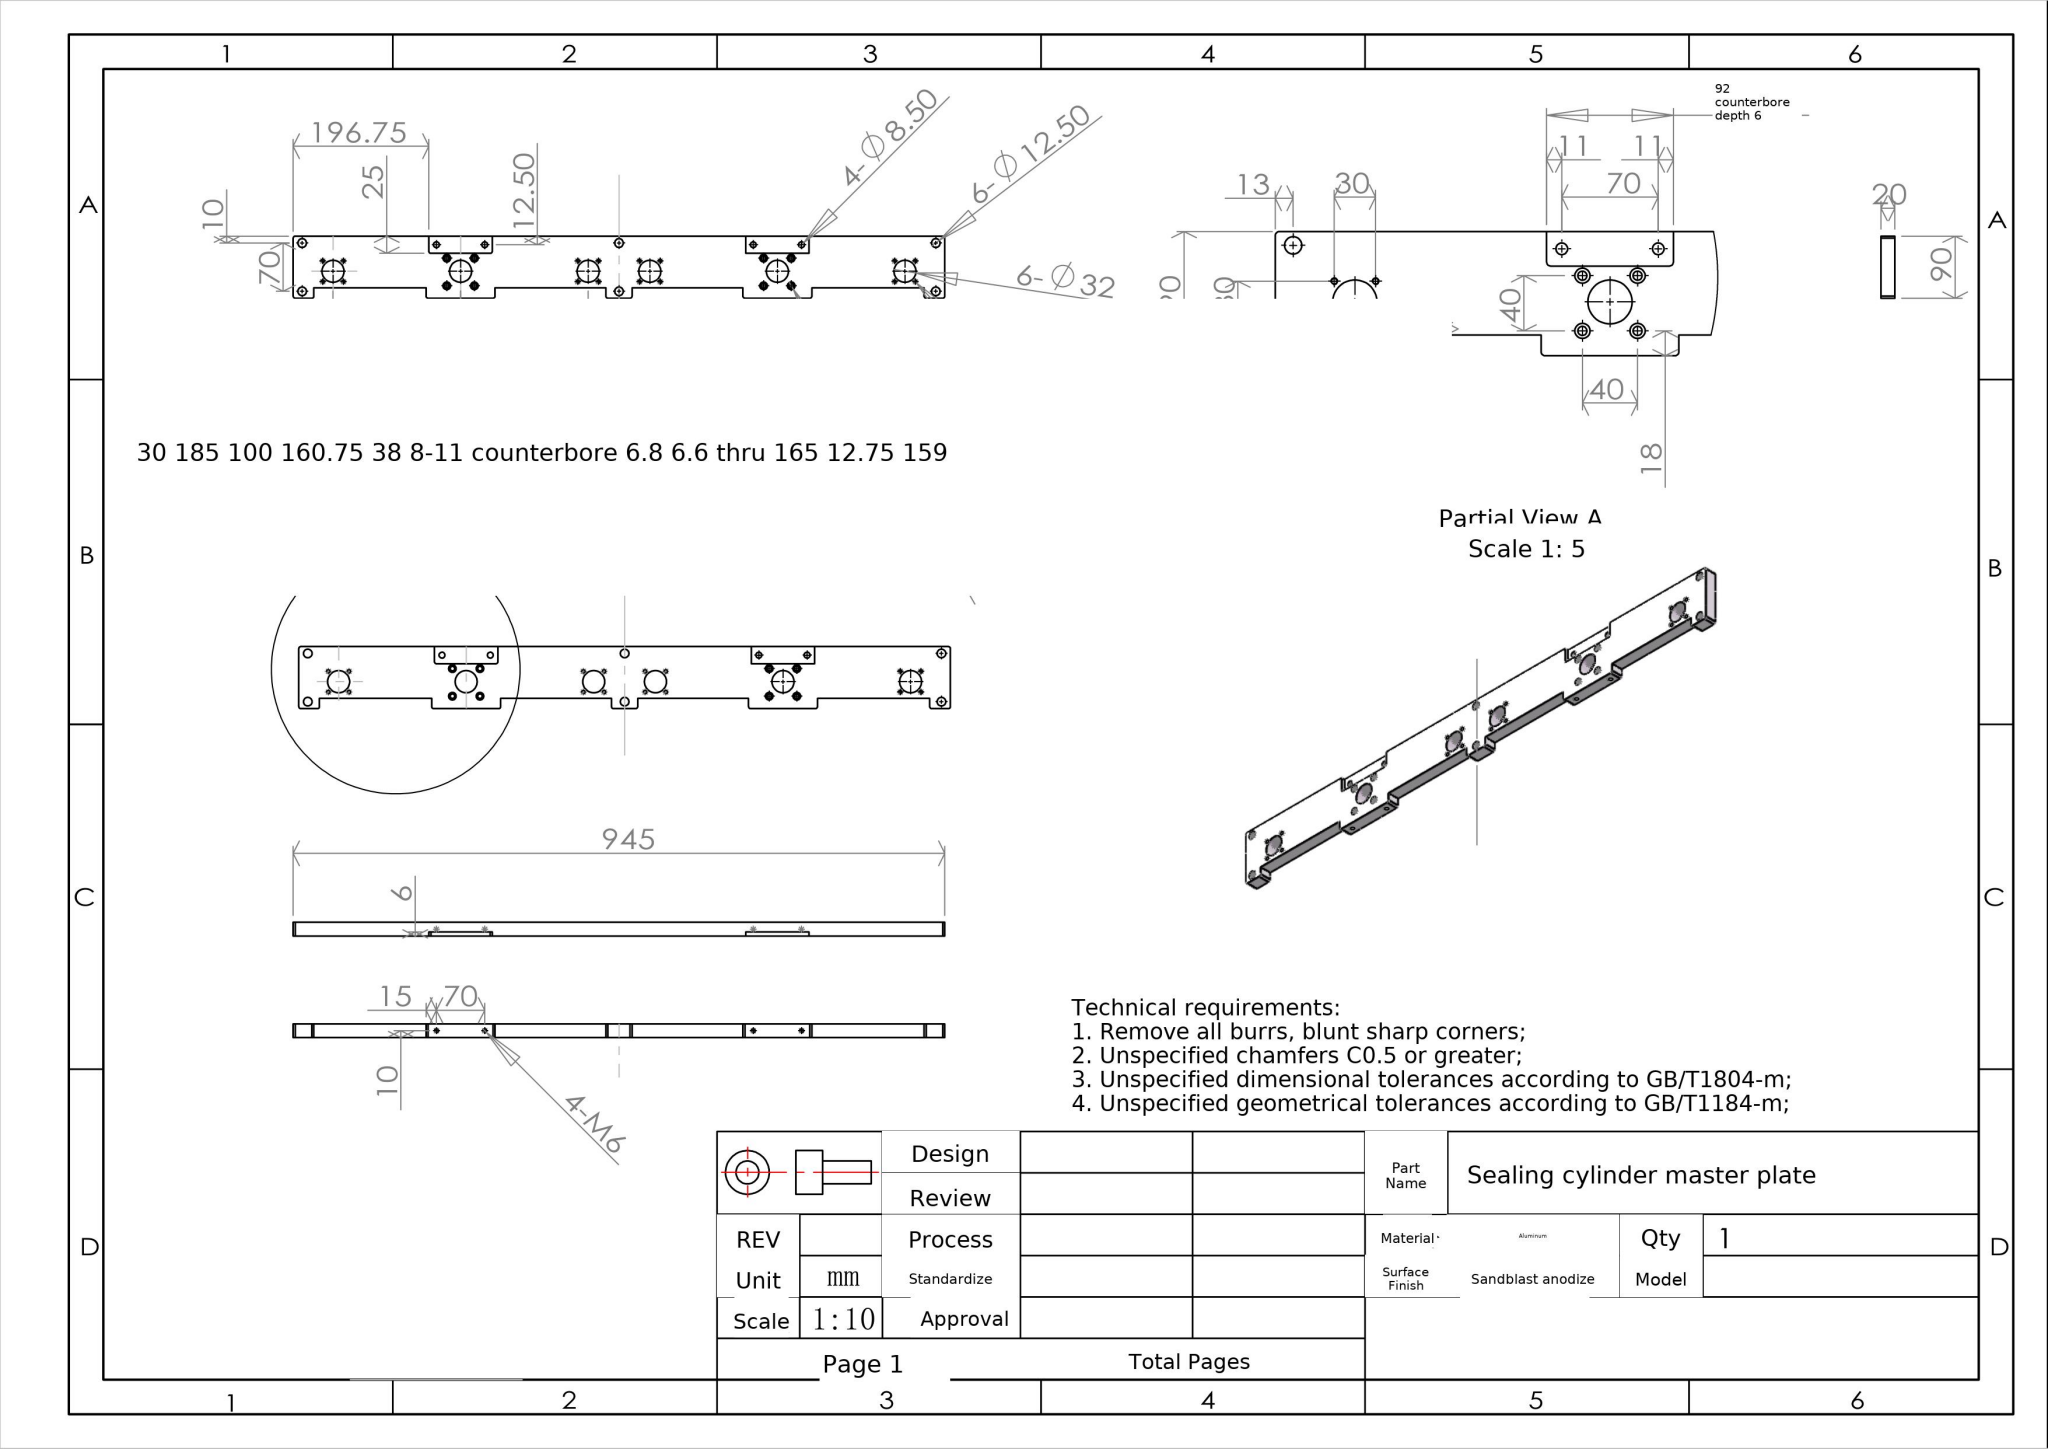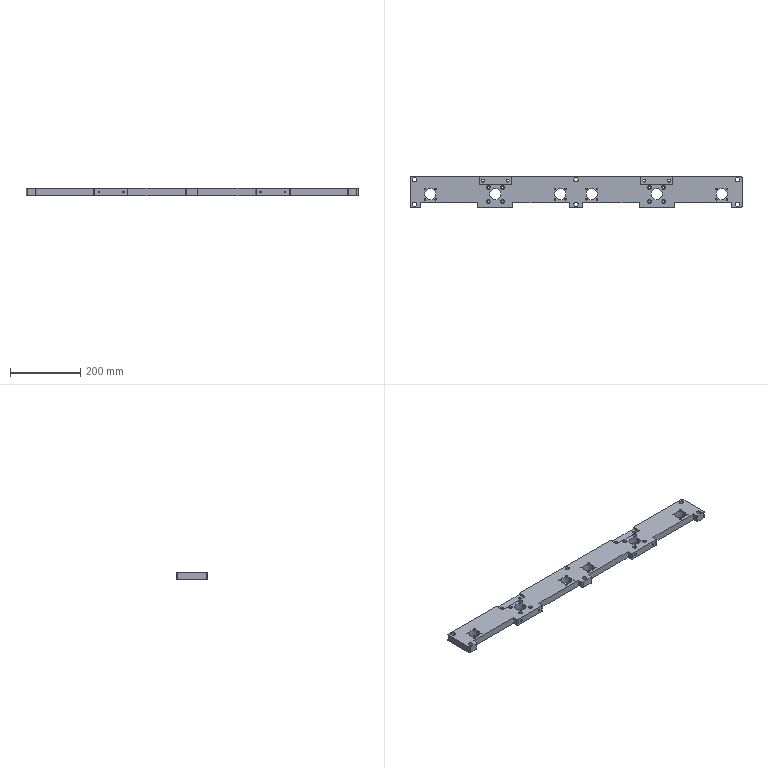Part | SolidWorks | mm | material Aluminum | 1 solid | 196 faces | box 945 x 90 x 20 mm | volume 1351604 mm3 | cylinder 118 | cone 40 | plane 38 | commonest cylinder face diameters 4.2 x32 11 x16 6.6 x16 6 x14 12.5 x12 32 x12 8.5 x8 5 x8
build123d program:
from build123d import *

# Parameters (mm, degrees)
BOSS_EXTRUDE1_DEPTH                                  = 20
SKETCH3_R                                            = 16
SKETCH3_R_2                                          = 6.25
CUT_EXTRUDE1_DEPTH                                   = 20
HOLE_SIZE_ACCORDING_TO_HEX_SOCKET_HEAD_C_D           = 6.6
HOLE_SIZE_ACCORDING_TO_HEX_SOCKET_HEAD_C_CBORE_D     = 11
HOLE_SIZE_ACCORDING_TO_HEX_SOCKET_HEAD_C_CBORE_DEPTH = 6.8
M5_TAPPED_HOLE2_D                                    = 4.2
M5_TAPPED_HOLE2_DEPTH                                = 12.4
M5_TAPPED_HOLE2_TIP                                  = 1.262
FILLET1_R                                            = 3
M6_TAPPED_HOLE2_D                                    = 5
M6_TAPPED_HOLE2_DEPTH                                = 15
M6_TAPPED_HOLE2_TIP                                  = 1.502
SKETCH12_W                                           = 92
SKETCH12_H                                           = 25
CUT_EXTRUDE2_DEPTH                                   = 6
SKETCH13_W                                           = 92
SKETCH13_H                                           = 25
CUT_EXTRUDE3_DEPTH                                   = 6
SKETCH14_R                                           = 4.25
CUT_EXTRUDE4_DEPTH                                   = 950.379
FILLET2_R                                            = 3


with BuildPart() as part:
    # Sketch1 → Boss-Extrude1 (new body)
    with BuildSketch(Plane.XY):
        Polygon((0, 0), (0, -90), (30, -90), (30, -75), (192.75, -75), (192.75, -90), (292.75, -90), (292.75, -75), (453.5, -75), (453.5, -90), (491.5, -90), (491.5, -75), (652.25, -75), (652.25, -90), (752.25, -90), (752.25, -75), (915, -75), (915, -90), (945, -90), (945, 0), align=None)
    extrude(amount=BOSS_EXTRUDE1_DEPTH)

    # Sketch3 → Cut-Extrude1 (cut)
    with BuildSketch(Plane.XY.offset(20)):
        with Locations((57.75, -51)):
            Circle(SKETCH3_R)
        with Locations((242.75, -51)):
            Circle(SKETCH3_R)
        with Locations((427.75, -51)):
            Circle(SKETCH3_R)
        with Locations((517.25, -51)):
            Circle(SKETCH3_R)
        with Locations((702.25, -51)):
            Circle(SKETCH3_R)
        with Locations((887.25, -51)):
            Circle(SKETCH3_R)
        with Locations((13, -10)):
            Circle(SKETCH3_R_2)
        with Locations((13, -80)):
            Circle(SKETCH3_R_2)
        with Locations((472.5, -10)):
            Circle(SKETCH3_R_2)
        with Locations((472.5, -80)):
            Circle(SKETCH3_R_2)
        with Locations((932, -10)):
            Circle(SKETCH3_R_2)
        with Locations((932, -80)):
            Circle(SKETCH3_R_2)
    extrude(amount=-CUT_EXTRUDE1_DEPTH, mode=Mode.SUBTRACT)

    # Hole Size according to Hex Socket Head C (through all)
    with Locations(Plane(origin=(222.75, -32, 20), x_dir=(1, 0, 0), z_dir=(0, 0, 1))):
        with Locations((0, 0), (0, -40), (40, -40), (40, 0), (459.5, 0), (459.5, -40), (499.5, -40), (499.5, 0)):
            CounterBoreHole(HOLE_SIZE_ACCORDING_TO_HEX_SOCKET_HEAD_C_D / 2, HOLE_SIZE_ACCORDING_TO_HEX_SOCKET_HEAD_C_CBORE_D / 2, HOLE_SIZE_ACCORDING_TO_HEX_SOCKET_HEAD_C_CBORE_DEPTH)

    # M5 Tapped Hole2
    with Locations(Plane(origin=(42.75, -36, 20), x_dir=(1, 0, 0), z_dir=(0, 0, 1))):
        with Locations((0, 0), (30, 0), (0, -30), (30, -30), (370, 0), (400, 0), (370, -30), (400, -30), (459.5, -30), (459.5, 0), (489.5, 0), (489.5, -30), (829.5, 0), (859.5, 0), (829.5, -30), (859.5, -30)):
            Hole(M5_TAPPED_HOLE2_D / 2, depth=M5_TAPPED_HOLE2_DEPTH)
            with Locations((0, 0, -(M5_TAPPED_HOLE2_DEPTH + M5_TAPPED_HOLE2_TIP / 2))):  # 118° drill point
                Cone(0, M5_TAPPED_HOLE2_D / 2, M5_TAPPED_HOLE2_TIP, mode=Mode.SUBTRACT)

    # Fillet1
    fillet1_edges = [part.edges().sort_by_distance(p)[0] for p in [
        (945, 0, 10),
        (945, -90, 10),
        (915, -90, 10),
        (752.25, -90, 10),
        (652.25, -90, 10),
        (491.5, -90, 10),
        (453.5, -90, 10),
        (292.75, -90, 10),
        (192.75, -90, 10),
        (30, -90, 10),
        (0, -90, 10),
        (0, 0, 10),
    ]]
    fillet(fillet1_edges, radius=FILLET1_R)

    # M6 Tapped Hole2
    with Locations(Plane(origin=(207.75, -90, 10), x_dir=(-1, 0, 0), z_dir=(0, -1, 0))):
        with Locations((0, 0), (-70, 0), (-459.5, 0), (-529.5, 0)):
            Hole(M6_TAPPED_HOLE2_D / 2, depth=M6_TAPPED_HOLE2_DEPTH)
            with Locations((0, 0, -(M6_TAPPED_HOLE2_DEPTH + M6_TAPPED_HOLE2_TIP / 2))):  # 118° drill point
                Cone(0, M6_TAPPED_HOLE2_D / 2, M6_TAPPED_HOLE2_TIP, mode=Mode.SUBTRACT)

    # Sketch12 → Cut-Extrude2 (cut)
    with BuildSketch(Plane.XY.offset(20)):
        with Locations((242.75, -12.5)):
            Rectangle(SKETCH12_W, SKETCH12_H)
    extrude(amount=-CUT_EXTRUDE2_DEPTH, mode=Mode.SUBTRACT)

    # Sketch13 → Cut-Extrude3 (cut)
    with BuildSketch(Plane.XY.offset(20)):
        with Locations((702.25, -12.5)):
            Rectangle(SKETCH13_W, SKETCH13_H)
    extrude(amount=-CUT_EXTRUDE3_DEPTH, mode=Mode.SUBTRACT)

    # Sketch14 → Cut-Extrude4 (cut, through all)
    with BuildSketch(Plane.XY.offset(14)):
        with Locations((207.75, -12.5)):
            Circle(SKETCH14_R)
        with Locations((277.75, -12.5)):
            Circle(SKETCH14_R)
        with Locations((667.25, -12.5)):
            Circle(SKETCH14_R)
        with Locations((737.25, -12.5)):
            Circle(SKETCH14_R)
    extrude(amount=-CUT_EXTRUDE4_DEPTH, mode=Mode.SUBTRACT)

    # Fillet2
    fillet2_edges = [part.edges().sort_by_distance(p)[0] for p in [
        (196.75, -25, 17),
        (288.75, -25, 17),
    ]]
    fillet(fillet2_edges, radius=FILLET2_R)


solid = part.part